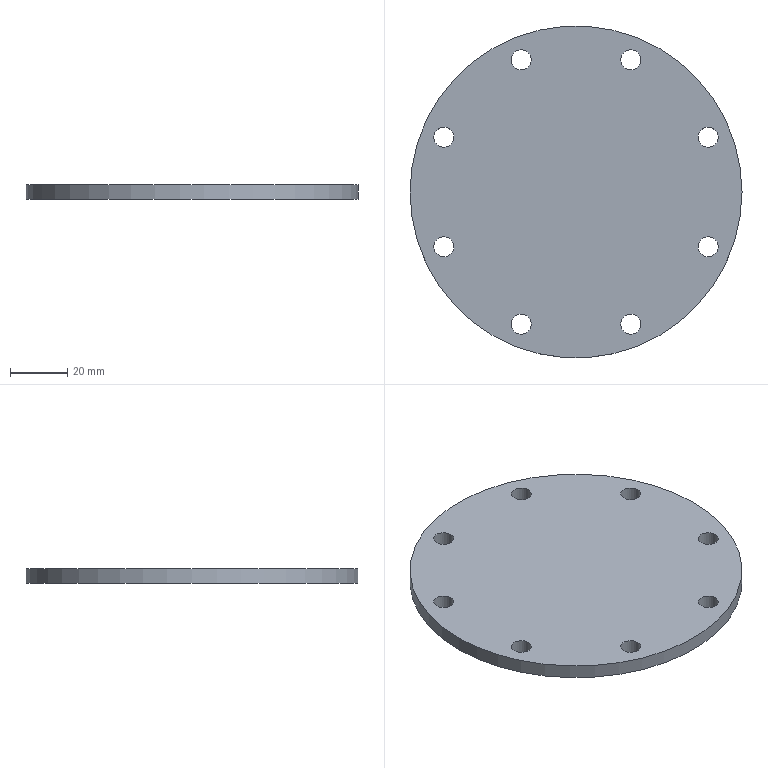Component | NX | CH3404-3 | 1 solid | 11 faces | box 116 x 116 x 5 mm | volume 51302 mm3 | cylinder 9 | plane 2 | commonest cylinder face diameters 7 x8 116 x1
STEP:
#1=CARTESIAN_POINT('',(0.,0.,0.));
#2=DIRECTION('',(0.,0.,1.));
#3=DIRECTION('',(1.,0.,0.));
#4=AXIS2_PLACEMENT_3D('',#1,#2,#3);
#5=CARTESIAN_POINT('',(58.531,0.1057,-1492.003));
#6=VERTEX_POINT('',#5);
#7=CARTESIAN_POINT('',(0.5308,0.1057,-1492.003));
#8=DIRECTION('',(0.,0.,1.));
#9=DIRECTION('',(1.,0.,0.));
#10=AXIS2_PLACEMENT_3D('',#7,#8,#9);
#11=CIRCLE('',#10,58.);
#12=CARTESIAN_POINT('',(0.5308,0.1057,-1492.003));
#13=DIRECTION('',(0.,0.,-1.));
#14=DIRECTION('',(-1.,0.,0.));
#15=AXIS2_PLACEMENT_3D('',#12,#13,#14);
#16=CYLINDRICAL_SURFACE('',#15,58.);
#17=CARTESIAN_POINT('',(9.425,0.));
#18=DIRECTION('',(-1.,0.));
#19=VECTOR('',#18,1.);
#20=LINE('',#17,#19);
#21=(GEOMETRIC_REPRESENTATION_CONTEXT(2)PARAMETRIC_REPRESENTATION_CONTEXT()REPRESENTATION_CONTEXT('',''));
#22=DEFINITIONAL_REPRESENTATION('',(#20),#21);
#23=PCURVE('',#16,#22);
#24=CARTESIAN_POINT('',(0.5308,0.1057,-1492.003));
#25=DIRECTION('',(0.,0.,1.));
#26=DIRECTION('',(1.,0.,0.));
#27=AXIS2_PLACEMENT_3D('',#24,#25,#26);
#28=PLANE('',#27);
#29=CARTESIAN_POINT('',(0.,0.));
#30=DIRECTION('',(1.,0.));
#31=AXIS2_PLACEMENT_2D('',#29,#30);
#32=CIRCLE('',#31,58.);
#33=(GEOMETRIC_REPRESENTATION_CONTEXT(2)PARAMETRIC_REPRESENTATION_CONTEXT()REPRESENTATION_CONTEXT('',''));
#34=DEFINITIONAL_REPRESENTATION('',(#32),#33);
#35=PCURVE('',#28,#34);
#36=SURFACE_CURVE('',#11,(#23,#35),.PCURVE_S1.);
#37=EDGE_CURVE('',#6,#6,#36,.T.);
#38=ORIENTED_EDGE('',*,*,#37,.F.);
#39=CARTESIAN_POINT('',(58.531,0.1057,-1497.003));
#40=VERTEX_POINT('',#39);
#41=CARTESIAN_POINT('',(58.531,0.1057,-1492.003));
#42=CARTESIAN_POINT('',(58.531,0.1057,-1497.003));
#43=B_SPLINE_CURVE_WITH_KNOTS('',1,(#41,#42),.UNSPECIFIED.,.F.,.F.,(2,2),(0.,5.),.PIECEWISE_BEZIER_KNOTS.);
#44=CARTESIAN_POINT('',(9.425,0.));
#45=DIRECTION('',(0.,1.));
#46=VECTOR('',#45,1.);
#47=LINE('',#44,#46);
#48=(GEOMETRIC_REPRESENTATION_CONTEXT(2)PARAMETRIC_REPRESENTATION_CONTEXT()REPRESENTATION_CONTEXT('',''));
#49=DEFINITIONAL_REPRESENTATION('',(#47),#48);
#50=PCURVE('',#16,#49);
#51=CARTESIAN_POINT('',(3.142,0.));
#52=DIRECTION('',(0.,1.));
#53=VECTOR('',#52,1.);
#54=LINE('',#51,#53);
#55=(GEOMETRIC_REPRESENTATION_CONTEXT(2)PARAMETRIC_REPRESENTATION_CONTEXT()REPRESENTATION_CONTEXT('',''));
#56=DEFINITIONAL_REPRESENTATION('',(#54),#55);
#57=PCURVE('',#16,#56);
#58=SEAM_CURVE('',#43,(#50,#57),.PCURVE_S1.);
#59=EDGE_CURVE('',#6,#40,#58,.T.);
#60=ORIENTED_EDGE('',*,*,#59,.T.);
#61=CARTESIAN_POINT('',(0.5308,0.1057,-1497.003));
#62=DIRECTION('',(0.,0.,1.));
#63=DIRECTION('',(1.,0.,0.));
#64=AXIS2_PLACEMENT_3D('',#61,#62,#63);
#65=CIRCLE('',#64,58.);
#66=CARTESIAN_POINT('',(9.425,5.));
#67=DIRECTION('',(-1.,0.));
#68=VECTOR('',#67,1.);
#69=LINE('',#66,#68);
#70=(GEOMETRIC_REPRESENTATION_CONTEXT(2)PARAMETRIC_REPRESENTATION_CONTEXT()REPRESENTATION_CONTEXT('',''));
#71=DEFINITIONAL_REPRESENTATION('',(#69),#70);
#72=PCURVE('',#16,#71);
#73=CARTESIAN_POINT('',(0.5308,0.1057,-1497.003));
#74=DIRECTION('',(0.,0.,1.));
#75=DIRECTION('',(1.,0.,0.));
#76=AXIS2_PLACEMENT_3D('',#73,#74,#75);
#77=PLANE('',#76);
#78=CARTESIAN_POINT('',(0.,0.));
#79=DIRECTION('',(1.,0.));
#80=AXIS2_PLACEMENT_2D('',#78,#79);
#81=CIRCLE('',#80,58.);
#82=(GEOMETRIC_REPRESENTATION_CONTEXT(2)PARAMETRIC_REPRESENTATION_CONTEXT()REPRESENTATION_CONTEXT('',''));
#83=DEFINITIONAL_REPRESENTATION('',(#81),#82);
#84=PCURVE('',#77,#83);
#85=SURFACE_CURVE('',#65,(#72,#84),.PCURVE_S1.);
#86=EDGE_CURVE('',#40,#40,#85,.T.);
#87=ORIENTED_EDGE('',*,*,#86,.T.);
#88=ORIENTED_EDGE('',*,*,#59,.F.);
#89=EDGE_LOOP('',(#38,#60,#87,#88));
#90=FACE_BOUND('',#89,.T.);
#91=ADVANCED_FACE('',(#90),#16,.T.);
#92=CARTESIAN_POINT('',(43.225,-19.028,-1492.003));
#93=VERTEX_POINT('',#92);
#94=CARTESIAN_POINT('',(46.725,-19.028,-1492.003));
#95=DIRECTION('',(0.,0.,-1.));
#96=DIRECTION('',(-1.,0.,0.));
#97=AXIS2_PLACEMENT_3D('',#94,#95,#96);
#98=CIRCLE('',#97,3.5);
#99=CARTESIAN_POINT('',(42.694,-19.134));
#100=CARTESIAN_POINT('',(42.694,-13.072));
#101=CARTESIAN_POINT('',(47.944,-16.103));
#102=CARTESIAN_POINT('',(53.194,-19.134));
#103=CARTESIAN_POINT('',(47.944,-22.165));
#104=CARTESIAN_POINT('',(42.694,-25.196));
#105=CARTESIAN_POINT('',(42.694,-19.134));
#106=(BOUNDED_CURVE()B_SPLINE_CURVE(2,(#99,#100,#101,#102,#103,#104,#105),.UNSPECIFIED.,.T.,.F.)B_SPLINE_CURVE_WITH_KNOTS((1,2,2,2,2,1),(-2.094,0.,2.094,4.189,6.283,8.378),.UNSPECIFIED.)CURVE()GEOMETRIC_REPRESENTATION_ITEM()RATIONAL_B_SPLINE_CURVE((1.,0.5,1.,0.5,1.,0.5,1.))REPRESENTATION_ITEM(''));
#107=(GEOMETRIC_REPRESENTATION_CONTEXT(2)PARAMETRIC_REPRESENTATION_CONTEXT()REPRESENTATION_CONTEXT('',''));
#108=DEFINITIONAL_REPRESENTATION('',(#106),#107);
#109=PCURVE('',#28,#108);
#110=CARTESIAN_POINT('',(46.725,-19.028,-1492.003));
#111=DIRECTION('',(0.,0.,-1.));
#112=DIRECTION('',(-1.,0.,0.));
#113=AXIS2_PLACEMENT_3D('',#110,#111,#112);
#114=CYLINDRICAL_SURFACE('',#113,3.5);
#115=CARTESIAN_POINT('',(0.,0.));
#116=DIRECTION('',(1.,0.));
#117=VECTOR('',#116,1.);
#118=LINE('',#115,#117);
#119=(GEOMETRIC_REPRESENTATION_CONTEXT(2)PARAMETRIC_REPRESENTATION_CONTEXT()REPRESENTATION_CONTEXT('',''));
#120=DEFINITIONAL_REPRESENTATION('',(#118),#119);
#121=PCURVE('',#114,#120);
#122=SURFACE_CURVE('',#98,(#109,#121),.PCURVE_S1.);
#123=EDGE_CURVE('',#93,#93,#122,.T.);
#124=ORIENTED_EDGE('',*,*,#123,.T.);
#125=EDGE_LOOP('',(#124));
#126=FACE_BOUND('',#125,.T.);
#127=CARTESIAN_POINT('',(16.165,-46.088,-1492.003));
#128=VERTEX_POINT('',#127);
#129=CARTESIAN_POINT('',(19.665,-46.088,-1492.003));
#130=DIRECTION('',(0.,0.,-1.));
#131=DIRECTION('',(-1.,0.,0.));
#132=AXIS2_PLACEMENT_3D('',#129,#130,#131);
#133=CIRCLE('',#132,3.5);
#134=CARTESIAN_POINT('',(15.634,-46.194));
#135=CARTESIAN_POINT('',(15.634,-40.132));
#136=CARTESIAN_POINT('',(20.884,-43.163));
#137=CARTESIAN_POINT('',(26.134,-46.194));
#138=CARTESIAN_POINT('',(20.884,-49.225));
#139=CARTESIAN_POINT('',(15.634,-52.256));
#140=CARTESIAN_POINT('',(15.634,-46.194));
#141=(BOUNDED_CURVE()B_SPLINE_CURVE(2,(#134,#135,#136,#137,#138,#139,#140),.UNSPECIFIED.,.T.,.F.)B_SPLINE_CURVE_WITH_KNOTS((1,2,2,2,2,1),(-2.094,0.,2.094,4.189,6.283,8.378),.UNSPECIFIED.)CURVE()GEOMETRIC_REPRESENTATION_ITEM()RATIONAL_B_SPLINE_CURVE((1.,0.5,1.,0.5,1.,0.5,1.))REPRESENTATION_ITEM(''));
#142=(GEOMETRIC_REPRESENTATION_CONTEXT(2)PARAMETRIC_REPRESENTATION_CONTEXT()REPRESENTATION_CONTEXT('',''));
#143=DEFINITIONAL_REPRESENTATION('',(#141),#142);
#144=PCURVE('',#28,#143);
#145=CARTESIAN_POINT('',(19.665,-46.088,-1492.003));
#146=DIRECTION('',(0.,0.,-1.));
#147=DIRECTION('',(-1.,0.,0.));
#148=AXIS2_PLACEMENT_3D('',#145,#146,#147);
#149=CYLINDRICAL_SURFACE('',#148,3.5);
#150=CARTESIAN_POINT('',(0.,0.));
#151=DIRECTION('',(1.,0.));
#152=VECTOR('',#151,1.);
#153=LINE('',#150,#152);
#154=(GEOMETRIC_REPRESENTATION_CONTEXT(2)PARAMETRIC_REPRESENTATION_CONTEXT()REPRESENTATION_CONTEXT('',''));
#155=DEFINITIONAL_REPRESENTATION('',(#153),#154);
#156=PCURVE('',#149,#155);
#157=SURFACE_CURVE('',#133,(#144,#156),.PCURVE_S1.);
#158=EDGE_CURVE('',#128,#128,#157,.T.);
#159=ORIENTED_EDGE('',*,*,#158,.T.);
#160=EDGE_LOOP('',(#159));
#161=FACE_BOUND('',#160,.T.);
#162=CARTESIAN_POINT('',(-22.103,-46.088,-1492.003));
#163=VERTEX_POINT('',#162);
#164=CARTESIAN_POINT('',(-18.603,-46.088,-1492.003));
#165=DIRECTION('',(0.,0.,-1.));
#166=DIRECTION('',(-1.,0.,0.));
#167=AXIS2_PLACEMENT_3D('',#164,#165,#166);
#168=CIRCLE('',#167,3.5);
#169=CARTESIAN_POINT('',(-22.634,-46.194));
#170=CARTESIAN_POINT('',(-22.634,-40.132));
#171=CARTESIAN_POINT('',(-17.384,-43.163));
#172=CARTESIAN_POINT('',(-12.134,-46.194));
#173=CARTESIAN_POINT('',(-17.384,-49.225));
#174=CARTESIAN_POINT('',(-22.634,-52.256));
#175=CARTESIAN_POINT('',(-22.634,-46.194));
#176=(BOUNDED_CURVE()B_SPLINE_CURVE(2,(#169,#170,#171,#172,#173,#174,#175),.UNSPECIFIED.,.T.,.F.)B_SPLINE_CURVE_WITH_KNOTS((1,2,2,2,2,1),(-2.094,0.,2.094,4.189,6.283,8.378),.UNSPECIFIED.)CURVE()GEOMETRIC_REPRESENTATION_ITEM()RATIONAL_B_SPLINE_CURVE((1.,0.5,1.,0.5,1.,0.5,1.))REPRESENTATION_ITEM(''));
#177=(GEOMETRIC_REPRESENTATION_CONTEXT(2)PARAMETRIC_REPRESENTATION_CONTEXT()REPRESENTATION_CONTEXT('',''));
#178=DEFINITIONAL_REPRESENTATION('',(#176),#177);
#179=PCURVE('',#28,#178);
#180=CARTESIAN_POINT('',(-18.603,-46.088,-1492.003));
#181=DIRECTION('',(0.,0.,-1.));
#182=DIRECTION('',(-1.,0.,0.));
#183=AXIS2_PLACEMENT_3D('',#180,#181,#182);
#184=CYLINDRICAL_SURFACE('',#183,3.5);
#185=CARTESIAN_POINT('',(0.,0.));
#186=DIRECTION('',(1.,0.));
#187=VECTOR('',#186,1.);
#188=LINE('',#185,#187);
#189=(GEOMETRIC_REPRESENTATION_CONTEXT(2)PARAMETRIC_REPRESENTATION_CONTEXT()REPRESENTATION_CONTEXT('',''));
#190=DEFINITIONAL_REPRESENTATION('',(#188),#189);
#191=PCURVE('',#184,#190);
#192=SURFACE_CURVE('',#168,(#179,#191),.PCURVE_S1.);
#193=EDGE_CURVE('',#163,#163,#192,.T.);
#194=ORIENTED_EDGE('',*,*,#193,.T.);
#195=EDGE_LOOP('',(#194));
#196=FACE_BOUND('',#195,.T.);
#197=CARTESIAN_POINT('',(-49.163,-19.028,-1492.003));
#198=VERTEX_POINT('',#197);
#199=CARTESIAN_POINT('',(-45.663,-19.028,-1492.003));
#200=DIRECTION('',(0.,0.,-1.));
#201=DIRECTION('',(-1.,0.,0.));
#202=AXIS2_PLACEMENT_3D('',#199,#200,#201);
#203=CIRCLE('',#202,3.5);
#204=CARTESIAN_POINT('',(-49.694,-19.134));
#205=CARTESIAN_POINT('',(-49.694,-13.072));
#206=CARTESIAN_POINT('',(-44.444,-16.103));
#207=CARTESIAN_POINT('',(-39.194,-19.134));
#208=CARTESIAN_POINT('',(-44.444,-22.165));
#209=CARTESIAN_POINT('',(-49.694,-25.196));
#210=CARTESIAN_POINT('',(-49.694,-19.134));
#211=(BOUNDED_CURVE()B_SPLINE_CURVE(2,(#204,#205,#206,#207,#208,#209,#210),.UNSPECIFIED.,.T.,.F.)B_SPLINE_CURVE_WITH_KNOTS((1,2,2,2,2,1),(-2.094,0.,2.094,4.189,6.283,8.378),.UNSPECIFIED.)CURVE()GEOMETRIC_REPRESENTATION_ITEM()RATIONAL_B_SPLINE_CURVE((1.,0.5,1.,0.5,1.,0.5,1.))REPRESENTATION_ITEM(''));
#212=(GEOMETRIC_REPRESENTATION_CONTEXT(2)PARAMETRIC_REPRESENTATION_CONTEXT()REPRESENTATION_CONTEXT('',''));
#213=DEFINITIONAL_REPRESENTATION('',(#211),#212);
#214=PCURVE('',#28,#213);
#215=CARTESIAN_POINT('',(-45.663,-19.028,-1492.003));
#216=DIRECTION('',(0.,0.,-1.));
#217=DIRECTION('',(-1.,0.,0.));
#218=AXIS2_PLACEMENT_3D('',#215,#216,#217);
#219=CYLINDRICAL_SURFACE('',#218,3.5);
#220=CARTESIAN_POINT('',(0.,0.));
#221=DIRECTION('',(1.,0.));
#222=VECTOR('',#221,1.);
#223=LINE('',#220,#222);
#224=(GEOMETRIC_REPRESENTATION_CONTEXT(2)PARAMETRIC_REPRESENTATION_CONTEXT()REPRESENTATION_CONTEXT('',''));
#225=DEFINITIONAL_REPRESENTATION('',(#223),#224);
#226=PCURVE('',#219,#225);
#227=SURFACE_CURVE('',#203,(#214,#226),.PCURVE_S1.);
#228=EDGE_CURVE('',#198,#198,#227,.T.);
#229=ORIENTED_EDGE('',*,*,#228,.T.);
#230=EDGE_LOOP('',(#229));
#231=FACE_BOUND('',#230,.T.);
#232=CARTESIAN_POINT('',(-49.163,19.24,-1492.003));
#233=VERTEX_POINT('',#232);
#234=CARTESIAN_POINT('',(-45.663,19.24,-1492.003));
#235=DIRECTION('',(0.,0.,-1.));
#236=DIRECTION('',(-1.,0.,0.));
#237=AXIS2_PLACEMENT_3D('',#234,#235,#236);
#238=CIRCLE('',#237,3.5);
#239=CARTESIAN_POINT('',(-49.694,19.134));
#240=CARTESIAN_POINT('',(-49.694,25.196));
#241=CARTESIAN_POINT('',(-44.444,22.165));
#242=CARTESIAN_POINT('',(-39.194,19.134));
#243=CARTESIAN_POINT('',(-44.444,16.103));
#244=CARTESIAN_POINT('',(-49.694,13.072));
#245=CARTESIAN_POINT('',(-49.694,19.134));
#246=(BOUNDED_CURVE()B_SPLINE_CURVE(2,(#239,#240,#241,#242,#243,#244,#245),.UNSPECIFIED.,.T.,.F.)B_SPLINE_CURVE_WITH_KNOTS((1,2,2,2,2,1),(-2.094,0.,2.094,4.189,6.283,8.378),.UNSPECIFIED.)CURVE()GEOMETRIC_REPRESENTATION_ITEM()RATIONAL_B_SPLINE_CURVE((1.,0.5,1.,0.5,1.,0.5,1.))REPRESENTATION_ITEM(''));
#247=(GEOMETRIC_REPRESENTATION_CONTEXT(2)PARAMETRIC_REPRESENTATION_CONTEXT()REPRESENTATION_CONTEXT('',''));
#248=DEFINITIONAL_REPRESENTATION('',(#246),#247);
#249=PCURVE('',#28,#248);
#250=CARTESIAN_POINT('',(-45.663,19.24,-1492.003));
#251=DIRECTION('',(0.,0.,-1.));
#252=DIRECTION('',(-1.,0.,0.));
#253=AXIS2_PLACEMENT_3D('',#250,#251,#252);
#254=CYLINDRICAL_SURFACE('',#253,3.5);
#255=CARTESIAN_POINT('',(0.,0.));
#256=DIRECTION('',(1.,0.));
#257=VECTOR('',#256,1.);
#258=LINE('',#255,#257);
#259=(GEOMETRIC_REPRESENTATION_CONTEXT(2)PARAMETRIC_REPRESENTATION_CONTEXT()REPRESENTATION_CONTEXT('',''));
#260=DEFINITIONAL_REPRESENTATION('',(#258),#259);
#261=PCURVE('',#254,#260);
#262=SURFACE_CURVE('',#238,(#249,#261),.PCURVE_S1.);
#263=EDGE_CURVE('',#233,#233,#262,.T.);
#264=ORIENTED_EDGE('',*,*,#263,.T.);
#265=EDGE_LOOP('',(#264));
#266=FACE_BOUND('',#265,.T.);
#267=CARTESIAN_POINT('',(-22.103,46.3,-1492.003));
#268=VERTEX_POINT('',#267);
#269=CARTESIAN_POINT('',(-18.603,46.3,-1492.003));
#270=DIRECTION('',(0.,0.,-1.));
#271=DIRECTION('',(-1.,0.,0.));
#272=AXIS2_PLACEMENT_3D('',#269,#270,#271);
#273=CIRCLE('',#272,3.5);
#274=CARTESIAN_POINT('',(-22.634,46.194));
#275=CARTESIAN_POINT('',(-22.634,52.256));
#276=CARTESIAN_POINT('',(-17.384,49.225));
#277=CARTESIAN_POINT('',(-12.134,46.194));
#278=CARTESIAN_POINT('',(-17.384,43.163));
#279=CARTESIAN_POINT('',(-22.634,40.132));
#280=CARTESIAN_POINT('',(-22.634,46.194));
#281=(BOUNDED_CURVE()B_SPLINE_CURVE(2,(#274,#275,#276,#277,#278,#279,#280),.UNSPECIFIED.,.T.,.F.)B_SPLINE_CURVE_WITH_KNOTS((1,2,2,2,2,1),(-2.094,0.,2.094,4.189,6.283,8.378),.UNSPECIFIED.)CURVE()GEOMETRIC_REPRESENTATION_ITEM()RATIONAL_B_SPLINE_CURVE((1.,0.5,1.,0.5,1.,0.5,1.))REPRESENTATION_ITEM(''));
#282=(GEOMETRIC_REPRESENTATION_CONTEXT(2)PARAMETRIC_REPRESENTATION_CONTEXT()REPRESENTATION_CONTEXT('',''));
#283=DEFINITIONAL_REPRESENTATION('',(#281),#282);
#284=PCURVE('',#28,#283);
#285=CARTESIAN_POINT('',(-18.603,46.3,-1492.003));
#286=DIRECTION('',(0.,0.,-1.));
#287=DIRECTION('',(-1.,0.,0.));
#288=AXIS2_PLACEMENT_3D('',#285,#286,#287);
#289=CYLINDRICAL_SURFACE('',#288,3.5);
#290=CARTESIAN_POINT('',(0.,0.));
#291=DIRECTION('',(1.,0.));
#292=VECTOR('',#291,1.);
#293=LINE('',#290,#292);
#294=(GEOMETRIC_REPRESENTATION_CONTEXT(2)PARAMETRIC_REPRESENTATION_CONTEXT()REPRESENTATION_CONTEXT('',''));
#295=DEFINITIONAL_REPRESENTATION('',(#293),#294);
#296=PCURVE('',#289,#295);
#297=SURFACE_CURVE('',#273,(#284,#296),.PCURVE_S1.);
#298=EDGE_CURVE('',#268,#268,#297,.T.);
#299=ORIENTED_EDGE('',*,*,#298,.T.);
#300=EDGE_LOOP('',(#299));
#301=FACE_BOUND('',#300,.T.);
#302=CARTESIAN_POINT('',(16.165,46.3,-1492.003));
#303=VERTEX_POINT('',#302);
#304=CARTESIAN_POINT('',(19.665,46.3,-1492.003));
#305=DIRECTION('',(0.,0.,-1.));
#306=DIRECTION('',(-1.,0.,0.));
#307=AXIS2_PLACEMENT_3D('',#304,#305,#306);
#308=CIRCLE('',#307,3.5);
#309=CARTESIAN_POINT('',(15.634,46.194));
#310=CARTESIAN_POINT('',(15.634,52.256));
#311=CARTESIAN_POINT('',(20.884,49.225));
#312=CARTESIAN_POINT('',(26.134,46.194));
#313=CARTESIAN_POINT('',(20.884,43.163));
#314=CARTESIAN_POINT('',(15.634,40.132));
#315=CARTESIAN_POINT('',(15.634,46.194));
#316=(BOUNDED_CURVE()B_SPLINE_CURVE(2,(#309,#310,#311,#312,#313,#314,#315),.UNSPECIFIED.,.T.,.F.)B_SPLINE_CURVE_WITH_KNOTS((1,2,2,2,2,1),(-2.094,0.,2.094,4.189,6.283,8.378),.UNSPECIFIED.)CURVE()GEOMETRIC_REPRESENTATION_ITEM()RATIONAL_B_SPLINE_CURVE((1.,0.5,1.,0.5,1.,0.5,1.))REPRESENTATION_ITEM(''));
#317=(GEOMETRIC_REPRESENTATION_CONTEXT(2)PARAMETRIC_REPRESENTATION_CONTEXT()REPRESENTATION_CONTEXT('',''));
#318=DEFINITIONAL_REPRESENTATION('',(#316),#317);
#319=PCURVE('',#28,#318);
#320=CARTESIAN_POINT('',(19.665,46.3,-1492.003));
#321=DIRECTION('',(0.,0.,-1.));
#322=DIRECTION('',(-1.,0.,0.));
#323=AXIS2_PLACEMENT_3D('',#320,#321,#322);
#324=CYLINDRICAL_SURFACE('',#323,3.5);
#325=CARTESIAN_POINT('',(0.,0.));
#326=DIRECTION('',(1.,0.));
#327=VECTOR('',#326,1.);
#328=LINE('',#325,#327);
#329=(GEOMETRIC_REPRESENTATION_CONTEXT(2)PARAMETRIC_REPRESENTATION_CONTEXT()REPRESENTATION_CONTEXT('',''));
#330=DEFINITIONAL_REPRESENTATION('',(#328),#329);
#331=PCURVE('',#324,#330);
#332=SURFACE_CURVE('',#308,(#319,#331),.PCURVE_S1.);
#333=EDGE_CURVE('',#303,#303,#332,.T.);
#334=ORIENTED_EDGE('',*,*,#333,.T.);
#335=EDGE_LOOP('',(#334));
#336=FACE_BOUND('',#335,.T.);
#337=CARTESIAN_POINT('',(43.225,19.24,-1492.003));
#338=VERTEX_POINT('',#337);
#339=CARTESIAN_POINT('',(46.725,19.24,-1492.003));
#340=DIRECTION('',(0.,0.,-1.));
#341=DIRECTION('',(-1.,0.,0.));
#342=AXIS2_PLACEMENT_3D('',#339,#340,#341);
#343=CIRCLE('',#342,3.5);
#344=CARTESIAN_POINT('',(42.694,19.134));
#345=CARTESIAN_POINT('',(42.694,25.196));
#346=CARTESIAN_POINT('',(47.944,22.165));
#347=CARTESIAN_POINT('',(53.194,19.134));
#348=CARTESIAN_POINT('',(47.944,16.103));
#349=CARTESIAN_POINT('',(42.694,13.072));
#350=CARTESIAN_POINT('',(42.694,19.134));
#351=(BOUNDED_CURVE()B_SPLINE_CURVE(2,(#344,#345,#346,#347,#348,#349,#350),.UNSPECIFIED.,.T.,.F.)B_SPLINE_CURVE_WITH_KNOTS((1,2,2,2,2,1),(-2.094,0.,2.094,4.189,6.283,8.378),.UNSPECIFIED.)CURVE()GEOMETRIC_REPRESENTATION_ITEM()RATIONAL_B_SPLINE_CURVE((1.,0.5,1.,0.5,1.,0.5,1.))REPRESENTATION_ITEM(''));
#352=(GEOMETRIC_REPRESENTATION_CONTEXT(2)PARAMETRIC_REPRESENTATION_CONTEXT()REPRESENTATION_CONTEXT('',''));
#353=DEFINITIONAL_REPRESENTATION('',(#351),#352);
#354=PCURVE('',#28,#353);
#355=CARTESIAN_POINT('',(46.725,19.24,-1492.003));
#356=DIRECTION('',(0.,0.,-1.));
#357=DIRECTION('',(-1.,0.,0.));
#358=AXIS2_PLACEMENT_3D('',#355,#356,#357);
#359=CYLINDRICAL_SURFACE('',#358,3.5);
#360=CARTESIAN_POINT('',(0.,0.));
#361=DIRECTION('',(1.,0.));
#362=VECTOR('',#361,1.);
#363=LINE('',#360,#362);
#364=(GEOMETRIC_REPRESENTATION_CONTEXT(2)PARAMETRIC_REPRESENTATION_CONTEXT()REPRESENTATION_CONTEXT('',''));
#365=DEFINITIONAL_REPRESENTATION('',(#363),#364);
#366=PCURVE('',#359,#365);
#367=SURFACE_CURVE('',#343,(#354,#366),.PCURVE_S1.);
#368=EDGE_CURVE('',#338,#338,#367,.T.);
#369=ORIENTED_EDGE('',*,*,#368,.T.);
#370=EDGE_LOOP('',(#369));
#371=FACE_BOUND('',#370,.T.);
#372=ORIENTED_EDGE('',*,*,#37,.T.);
#373=EDGE_LOOP('',(#372));
#374=FACE_BOUND('',#373,.T.);
#375=ADVANCED_FACE('',(#126,#161,#196,#231,#266,#301,#336,#371,#374),#28,.T.);
#376=CARTESIAN_POINT('',(50.225,-19.028,-1497.003));
#377=VERTEX_POINT('',#376);
#378=CARTESIAN_POINT('',(43.225,-19.028,-1497.003));
#379=VERTEX_POINT('',#378);
#380=CARTESIAN_POINT('',(46.725,-19.028,-1497.003));
#381=DIRECTION('',(0.,0.,1.));
#382=DIRECTION('',(1.,0.,0.));
#383=AXIS2_PLACEMENT_3D('',#380,#381,#382);
#384=CIRCLE('',#383,3.5);
#385=CARTESIAN_POINT('',(46.194,-19.134));
#386=DIRECTION('',(1.,0.));
#387=AXIS2_PLACEMENT_2D('',#385,#386);
#388=CIRCLE('',#387,3.5);
#389=(GEOMETRIC_REPRESENTATION_CONTEXT(2)PARAMETRIC_REPRESENTATION_CONTEXT()REPRESENTATION_CONTEXT('',''));
#390=DEFINITIONAL_REPRESENTATION('',(#388),#389);
#391=PCURVE('',#77,#390);
#392=CARTESIAN_POINT('',(3.142,5.));
#393=DIRECTION('',(-1.,0.));
#394=VECTOR('',#393,1.);
#395=LINE('',#392,#394);
#396=(GEOMETRIC_REPRESENTATION_CONTEXT(2)PARAMETRIC_REPRESENTATION_CONTEXT()REPRESENTATION_CONTEXT('',''));
#397=DEFINITIONAL_REPRESENTATION('',(#395),#396);
#398=PCURVE('',#114,#397);
#399=SURFACE_CURVE('',#384,(#391,#398),.PCURVE_S1.);
#400=EDGE_CURVE('',#377,#379,#399,.T.);
#401=ORIENTED_EDGE('',*,*,#400,.T.);
#402=CARTESIAN_POINT('',(46.725,-19.028,-1497.003));
#403=DIRECTION('',(0.,0.,1.));
#404=DIRECTION('',(1.,0.,0.));
#405=AXIS2_PLACEMENT_3D('',#402,#403,#404);
#406=CIRCLE('',#405,3.5);
#407=CARTESIAN_POINT('',(46.194,-19.134));
#408=DIRECTION('',(1.,0.));
#409=AXIS2_PLACEMENT_2D('',#407,#408);
#410=CIRCLE('',#409,3.5);
#411=(GEOMETRIC_REPRESENTATION_CONTEXT(2)PARAMETRIC_REPRESENTATION_CONTEXT()REPRESENTATION_CONTEXT('',''));
#412=DEFINITIONAL_REPRESENTATION('',(#410),#411);
#413=PCURVE('',#77,#412);
#414=CARTESIAN_POINT('',(9.425,5.));
#415=DIRECTION('',(-1.,0.));
#416=VECTOR('',#415,1.);
#417=LINE('',#414,#416);
#418=(GEOMETRIC_REPRESENTATION_CONTEXT(2)PARAMETRIC_REPRESENTATION_CONTEXT()REPRESENTATION_CONTEXT('',''));
#419=DEFINITIONAL_REPRESENTATION('',(#417),#418);
#420=PCURVE('',#114,#419);
#421=SURFACE_CURVE('',#406,(#413,#420),.PCURVE_S1.);
#422=EDGE_CURVE('',#379,#377,#421,.T.);
#423=ORIENTED_EDGE('',*,*,#422,.T.);
#424=EDGE_LOOP('',(#401,#423));
#425=FACE_BOUND('',#424,.T.);
#426=CARTESIAN_POINT('',(23.165,-46.088,-1497.003));
#427=VERTEX_POINT('',#426);
#428=CARTESIAN_POINT('',(16.165,-46.088,-1497.003));
#429=VERTEX_POINT('',#428);
#430=CARTESIAN_POINT('',(19.665,-46.088,-1497.003));
#431=DIRECTION('',(0.,0.,1.));
#432=DIRECTION('',(1.,0.,0.));
#433=AXIS2_PLACEMENT_3D('',#430,#431,#432);
#434=CIRCLE('',#433,3.5);
#435=CARTESIAN_POINT('',(19.134,-46.194));
#436=DIRECTION('',(1.,0.));
#437=AXIS2_PLACEMENT_2D('',#435,#436);
#438=CIRCLE('',#437,3.5);
#439=(GEOMETRIC_REPRESENTATION_CONTEXT(2)PARAMETRIC_REPRESENTATION_CONTEXT()REPRESENTATION_CONTEXT('',''));
#440=DEFINITIONAL_REPRESENTATION('',(#438),#439);
#441=PCURVE('',#77,#440);
#442=CARTESIAN_POINT('',(3.142,5.));
#443=DIRECTION('',(-1.,0.));
#444=VECTOR('',#443,1.);
#445=LINE('',#442,#444);
#446=(GEOMETRIC_REPRESENTATION_CONTEXT(2)PARAMETRIC_REPRESENTATION_CONTEXT()REPRESENTATION_CONTEXT('',''));
#447=DEFINITIONAL_REPRESENTATION('',(#445),#446);
#448=PCURVE('',#149,#447);
#449=SURFACE_CURVE('',#434,(#441,#448),.PCURVE_S1.);
#450=EDGE_CURVE('',#427,#429,#449,.T.);
#451=ORIENTED_EDGE('',*,*,#450,.T.);
#452=CARTESIAN_POINT('',(19.665,-46.088,-1497.003));
#453=DIRECTION('',(0.,0.,1.));
#454=DIRECTION('',(1.,0.,0.));
#455=AXIS2_PLACEMENT_3D('',#452,#453,#454);
#456=CIRCLE('',#455,3.5);
#457=CARTESIAN_POINT('',(19.134,-46.194));
#458=DIRECTION('',(1.,0.));
#459=AXIS2_PLACEMENT_2D('',#457,#458);
#460=CIRCLE('',#459,3.5);
#461=(GEOMETRIC_REPRESENTATION_CONTEXT(2)PARAMETRIC_REPRESENTATION_CONTEXT()REPRESENTATION_CONTEXT('',''));
#462=DEFINITIONAL_REPRESENTATION('',(#460),#461);
#463=PCURVE('',#77,#462);
#464=CARTESIAN_POINT('',(9.425,5.));
#465=DIRECTION('',(-1.,0.));
#466=VECTOR('',#465,1.);
#467=LINE('',#464,#466);
#468=(GEOMETRIC_REPRESENTATION_CONTEXT(2)PARAMETRIC_REPRESENTATION_CONTEXT()REPRESENTATION_CONTEXT('',''));
#469=DEFINITIONAL_REPRESENTATION('',(#467),#468);
#470=PCURVE('',#149,#469);
#471=SURFACE_CURVE('',#456,(#463,#470),.PCURVE_S1.);
#472=EDGE_CURVE('',#429,#427,#471,.T.);
#473=ORIENTED_EDGE('',*,*,#472,.T.);
#474=EDGE_LOOP('',(#451,#473));
#475=FACE_BOUND('',#474,.T.);
#476=CARTESIAN_POINT('',(-15.103,-46.088,-1497.003));
#477=VERTEX_POINT('',#476);
#478=CARTESIAN_POINT('',(-22.103,-46.088,-1497.003));
#479=VERTEX_POINT('',#478);
#480=CARTESIAN_POINT('',(-18.603,-46.088,-1497.003));
#481=DIRECTION('',(0.,0.,1.));
#482=DIRECTION('',(1.,0.,0.));
#483=AXIS2_PLACEMENT_3D('',#480,#481,#482);
#484=CIRCLE('',#483,3.5);
#485=CARTESIAN_POINT('',(-19.134,-46.194));
#486=DIRECTION('',(1.,0.));
#487=AXIS2_PLACEMENT_2D('',#485,#486);
#488=CIRCLE('',#487,3.5);
#489=(GEOMETRIC_REPRESENTATION_CONTEXT(2)PARAMETRIC_REPRESENTATION_CONTEXT()REPRESENTATION_CONTEXT('',''));
#490=DEFINITIONAL_REPRESENTATION('',(#488),#489);
#491=PCURVE('',#77,#490);
#492=CARTESIAN_POINT('',(3.142,5.));
#493=DIRECTION('',(-1.,0.));
#494=VECTOR('',#493,1.);
#495=LINE('',#492,#494);
#496=(GEOMETRIC_REPRESENTATION_CONTEXT(2)PARAMETRIC_REPRESENTATION_CONTEXT()REPRESENTATION_CONTEXT('',''));
#497=DEFINITIONAL_REPRESENTATION('',(#495),#496);
#498=PCURVE('',#184,#497);
#499=SURFACE_CURVE('',#484,(#491,#498),.PCURVE_S1.);
#500=EDGE_CURVE('',#477,#479,#499,.T.);
#501=ORIENTED_EDGE('',*,*,#500,.T.);
#502=CARTESIAN_POINT('',(-18.603,-46.088,-1497.003));
#503=DIRECTION('',(0.,0.,1.));
#504=DIRECTION('',(1.,0.,0.));
#505=AXIS2_PLACEMENT_3D('',#502,#503,#504);
#506=CIRCLE('',#505,3.5);
#507=CARTESIAN_POINT('',(-19.134,-46.194));
#508=DIRECTION('',(1.,0.));
#509=AXIS2_PLACEMENT_2D('',#507,#508);
#510=CIRCLE('',#509,3.5);
#511=(GEOMETRIC_REPRESENTATION_CONTEXT(2)PARAMETRIC_REPRESENTATION_CONTEXT()REPRESENTATION_CONTEXT('',''));
#512=DEFINITIONAL_REPRESENTATION('',(#510),#511);
#513=PCURVE('',#77,#512);
#514=CARTESIAN_POINT('',(9.425,5.));
#515=DIRECTION('',(-1.,0.));
#516=VECTOR('',#515,1.);
#517=LINE('',#514,#516);
#518=(GEOMETRIC_REPRESENTATION_CONTEXT(2)PARAMETRIC_REPRESENTATION_CONTEXT()REPRESENTATION_CONTEXT('',''));
#519=DEFINITIONAL_REPRESENTATION('',(#517),#518);
#520=PCURVE('',#184,#519);
#521=SURFACE_CURVE('',#506,(#513,#520),.PCURVE_S1.);
#522=EDGE_CURVE('',#479,#477,#521,.T.);
#523=ORIENTED_EDGE('',*,*,#522,.T.);
#524=EDGE_LOOP('',(#501,#523));
#525=FACE_BOUND('',#524,.T.);
#526=CARTESIAN_POINT('',(-42.163,-19.028,-1497.003));
#527=VERTEX_POINT('',#526);
#528=CARTESIAN_POINT('',(-49.163,-19.028,-1497.003));
#529=VERTEX_POINT('',#528);
#530=CARTESIAN_POINT('',(-45.663,-19.028,-1497.003));
#531=DIRECTION('',(0.,0.,1.));
#532=DIRECTION('',(1.,0.,0.));
#533=AXIS2_PLACEMENT_3D('',#530,#531,#532);
#534=CIRCLE('',#533,3.5);
#535=CARTESIAN_POINT('',(-46.194,-19.134));
#536=DIRECTION('',(1.,0.));
#537=AXIS2_PLACEMENT_2D('',#535,#536);
#538=CIRCLE('',#537,3.5);
#539=(GEOMETRIC_REPRESENTATION_CONTEXT(2)PARAMETRIC_REPRESENTATION_CONTEXT()REPRESENTATION_CONTEXT('',''));
#540=DEFINITIONAL_REPRESENTATION('',(#538),#539);
#541=PCURVE('',#77,#540);
#542=CARTESIAN_POINT('',(3.142,5.));
#543=DIRECTION('',(-1.,0.));
#544=VECTOR('',#543,1.);
#545=LINE('',#542,#544);
#546=(GEOMETRIC_REPRESENTATION_CONTEXT(2)PARAMETRIC_REPRESENTATION_CONTEXT()REPRESENTATION_CONTEXT('',''));
#547=DEFINITIONAL_REPRESENTATION('',(#545),#546);
#548=PCURVE('',#219,#547);
#549=SURFACE_CURVE('',#534,(#541,#548),.PCURVE_S1.);
#550=EDGE_CURVE('',#527,#529,#549,.T.);
#551=ORIENTED_EDGE('',*,*,#550,.T.);
#552=CARTESIAN_POINT('',(-45.663,-19.028,-1497.003));
#553=DIRECTION('',(0.,0.,1.));
#554=DIRECTION('',(1.,0.,0.));
#555=AXIS2_PLACEMENT_3D('',#552,#553,#554);
#556=CIRCLE('',#555,3.5);
#557=CARTESIAN_POINT('',(-46.194,-19.134));
#558=DIRECTION('',(1.,0.));
#559=AXIS2_PLACEMENT_2D('',#557,#558);
#560=CIRCLE('',#559,3.5);
#561=(GEOMETRIC_REPRESENTATION_CONTEXT(2)PARAMETRIC_REPRESENTATION_CONTEXT()REPRESENTATION_CONTEXT('',''));
#562=DEFINITIONAL_REPRESENTATION('',(#560),#561);
#563=PCURVE('',#77,#562);
#564=CARTESIAN_POINT('',(9.425,5.));
#565=DIRECTION('',(-1.,0.));
#566=VECTOR('',#565,1.);
#567=LINE('',#564,#566);
#568=(GEOMETRIC_REPRESENTATION_CONTEXT(2)PARAMETRIC_REPRESENTATION_CONTEXT()REPRESENTATION_CONTEXT('',''));
#569=DEFINITIONAL_REPRESENTATION('',(#567),#568);
#570=PCURVE('',#219,#569);
#571=SURFACE_CURVE('',#556,(#563,#570),.PCURVE_S1.);
#572=EDGE_CURVE('',#529,#527,#571,.T.);
#573=ORIENTED_EDGE('',*,*,#572,.T.);
#574=EDGE_LOOP('',(#551,#573));
#575=FACE_BOUND('',#574,.T.);
#576=CARTESIAN_POINT('',(-42.163,19.24,-1497.003));
#577=VERTEX_POINT('',#576);
#578=CARTESIAN_POINT('',(-49.163,19.24,-1497.003));
#579=VERTEX_POINT('',#578);
#580=CARTESIAN_POINT('',(-45.663,19.24,-1497.003));
#581=DIRECTION('',(0.,0.,1.));
#582=DIRECTION('',(1.,0.,0.));
#583=AXIS2_PLACEMENT_3D('',#580,#581,#582);
#584=CIRCLE('',#583,3.5);
#585=CARTESIAN_POINT('',(-46.194,19.134));
#586=DIRECTION('',(1.,0.));
#587=AXIS2_PLACEMENT_2D('',#585,#586);
#588=CIRCLE('',#587,3.5);
#589=(GEOMETRIC_REPRESENTATION_CONTEXT(2)PARAMETRIC_REPRESENTATION_CONTEXT()REPRESENTATION_CONTEXT('',''));
#590=DEFINITIONAL_REPRESENTATION('',(#588),#589);
#591=PCURVE('',#77,#590);
#592=CARTESIAN_POINT('',(3.142,5.));
#593=DIRECTION('',(-1.,0.));
#594=VECTOR('',#593,1.);
#595=LINE('',#592,#594);
#596=(GEOMETRIC_REPRESENTATION_CONTEXT(2)PARAMETRIC_REPRESENTATION_CONTEXT()REPRESENTATION_CONTEXT('',''));
#597=DEFINITIONAL_REPRESENTATION('',(#595),#596);
#598=PCURVE('',#254,#597);
#599=SURFACE_CURVE('',#584,(#591,#598),.PCURVE_S1.);
#600=EDGE_CURVE('',#577,#579,#599,.T.);
#601=ORIENTED_EDGE('',*,*,#600,.T.);
#602=CARTESIAN_POINT('',(-45.663,19.24,-1497.003));
#603=DIRECTION('',(0.,0.,1.));
#604=DIRECTION('',(1.,0.,0.));
#605=AXIS2_PLACEMENT_3D('',#602,#603,#604);
#606=CIRCLE('',#605,3.5);
#607=CARTESIAN_POINT('',(-46.194,19.134));
#608=DIRECTION('',(1.,0.));
#609=AXIS2_PLACEMENT_2D('',#607,#608);
#610=CIRCLE('',#609,3.5);
#611=(GEOMETRIC_REPRESENTATION_CONTEXT(2)PARAMETRIC_REPRESENTATION_CONTEXT()REPRESENTATION_CONTEXT('',''));
#612=DEFINITIONAL_REPRESENTATION('',(#610),#611);
#613=PCURVE('',#77,#612);
#614=CARTESIAN_POINT('',(9.425,5.));
#615=DIRECTION('',(-1.,0.));
#616=VECTOR('',#615,1.);
#617=LINE('',#614,#616);
#618=(GEOMETRIC_REPRESENTATION_CONTEXT(2)PARAMETRIC_REPRESENTATION_CONTEXT()REPRESENTATION_CONTEXT('',''));
#619=DEFINITIONAL_REPRESENTATION('',(#617),#618);
#620=PCURVE('',#254,#619);
#621=SURFACE_CURVE('',#606,(#613,#620),.PCURVE_S1.);
#622=EDGE_CURVE('',#579,#577,#621,.T.);
#623=ORIENTED_EDGE('',*,*,#622,.T.);
#624=EDGE_LOOP('',(#601,#623));
#625=FACE_BOUND('',#624,.T.);
#626=CARTESIAN_POINT('',(-15.103,46.3,-1497.003));
#627=VERTEX_POINT('',#626);
#628=CARTESIAN_POINT('',(-22.103,46.3,-1497.003));
#629=VERTEX_POINT('',#628);
#630=CARTESIAN_POINT('',(-18.603,46.3,-1497.003));
#631=DIRECTION('',(0.,0.,1.));
#632=DIRECTION('',(1.,0.,0.));
#633=AXIS2_PLACEMENT_3D('',#630,#631,#632);
#634=CIRCLE('',#633,3.5);
#635=CARTESIAN_POINT('',(-19.134,46.194));
#636=DIRECTION('',(1.,0.));
#637=AXIS2_PLACEMENT_2D('',#635,#636);
#638=CIRCLE('',#637,3.5);
#639=(GEOMETRIC_REPRESENTATION_CONTEXT(2)PARAMETRIC_REPRESENTATION_CONTEXT()REPRESENTATION_CONTEXT('',''));
#640=DEFINITIONAL_REPRESENTATION('',(#638),#639);
#641=PCURVE('',#77,#640);
#642=CARTESIAN_POINT('',(3.142,5.));
#643=DIRECTION('',(-1.,0.));
#644=VECTOR('',#643,1.);
#645=LINE('',#642,#644);
#646=(GEOMETRIC_REPRESENTATION_CONTEXT(2)PARAMETRIC_REPRESENTATION_CONTEXT()REPRESENTATION_CONTEXT('',''));
#647=DEFINITIONAL_REPRESENTATION('',(#645),#646);
#648=PCURVE('',#289,#647);
#649=SURFACE_CURVE('',#634,(#641,#648),.PCURVE_S1.);
#650=EDGE_CURVE('',#627,#629,#649,.T.);
#651=ORIENTED_EDGE('',*,*,#650,.T.);
#652=CARTESIAN_POINT('',(-18.603,46.3,-1497.003));
#653=DIRECTION('',(0.,0.,1.));
#654=DIRECTION('',(1.,0.,0.));
#655=AXIS2_PLACEMENT_3D('',#652,#653,#654);
#656=CIRCLE('',#655,3.5);
#657=CARTESIAN_POINT('',(-19.134,46.194));
#658=DIRECTION('',(1.,0.));
#659=AXIS2_PLACEMENT_2D('',#657,#658);
#660=CIRCLE('',#659,3.5);
#661=(GEOMETRIC_REPRESENTATION_CONTEXT(2)PARAMETRIC_REPRESENTATION_CONTEXT()REPRESENTATION_CONTEXT('',''));
#662=DEFINITIONAL_REPRESENTATION('',(#660),#661);
#663=PCURVE('',#77,#662);
#664=CARTESIAN_POINT('',(9.425,5.));
#665=DIRECTION('',(-1.,0.));
#666=VECTOR('',#665,1.);
#667=LINE('',#664,#666);
#668=(GEOMETRIC_REPRESENTATION_CONTEXT(2)PARAMETRIC_REPRESENTATION_CONTEXT()REPRESENTATION_CONTEXT('',''));
#669=DEFINITIONAL_REPRESENTATION('',(#667),#668);
#670=PCURVE('',#289,#669);
#671=SURFACE_CURVE('',#656,(#663,#670),.PCURVE_S1.);
#672=EDGE_CURVE('',#629,#627,#671,.T.);
#673=ORIENTED_EDGE('',*,*,#672,.T.);
#674=EDGE_LOOP('',(#651,#673));
#675=FACE_BOUND('',#674,.T.);
#676=CARTESIAN_POINT('',(23.165,46.3,-1497.003));
#677=VERTEX_POINT('',#676);
#678=CARTESIAN_POINT('',(16.165,46.3,-1497.003));
#679=VERTEX_POINT('',#678);
#680=CARTESIAN_POINT('',(19.665,46.3,-1497.003));
#681=DIRECTION('',(0.,0.,1.));
#682=DIRECTION('',(1.,0.,0.));
#683=AXIS2_PLACEMENT_3D('',#680,#681,#682);
#684=CIRCLE('',#683,3.5);
#685=CARTESIAN_POINT('',(19.134,46.194));
#686=DIRECTION('',(1.,0.));
#687=AXIS2_PLACEMENT_2D('',#685,#686);
#688=CIRCLE('',#687,3.5);
#689=(GEOMETRIC_REPRESENTATION_CONTEXT(2)PARAMETRIC_REPRESENTATION_CONTEXT()REPRESENTATION_CONTEXT('',''));
#690=DEFINITIONAL_REPRESENTATION('',(#688),#689);
#691=PCURVE('',#77,#690);
#692=CARTESIAN_POINT('',(3.142,5.));
#693=DIRECTION('',(-1.,0.));
#694=VECTOR('',#693,1.);
#695=LINE('',#692,#694);
#696=(GEOMETRIC_REPRESENTATION_CONTEXT(2)PARAMETRIC_REPRESENTATION_CONTEXT()REPRESENTATION_CONTEXT('',''));
#697=DEFINITIONAL_REPRESENTATION('',(#695),#696);
#698=PCURVE('',#324,#697);
#699=SURFACE_CURVE('',#684,(#691,#698),.PCURVE_S1.);
#700=EDGE_CURVE('',#677,#679,#699,.T.);
#701=ORIENTED_EDGE('',*,*,#700,.T.);
#702=CARTESIAN_POINT('',(19.665,46.3,-1497.003));
#703=DIRECTION('',(0.,0.,1.));
#704=DIRECTION('',(1.,0.,0.));
#705=AXIS2_PLACEMENT_3D('',#702,#703,#704);
#706=CIRCLE('',#705,3.5);
#707=CARTESIAN_POINT('',(19.134,46.194));
#708=DIRECTION('',(1.,0.));
#709=AXIS2_PLACEMENT_2D('',#707,#708);
#710=CIRCLE('',#709,3.5);
#711=(GEOMETRIC_REPRESENTATION_CONTEXT(2)PARAMETRIC_REPRESENTATION_CONTEXT()REPRESENTATION_CONTEXT('',''));
#712=DEFINITIONAL_REPRESENTATION('',(#710),#711);
#713=PCURVE('',#77,#712);
#714=CARTESIAN_POINT('',(9.425,5.));
#715=DIRECTION('',(-1.,0.));
#716=VECTOR('',#715,1.);
#717=LINE('',#714,#716);
#718=(GEOMETRIC_REPRESENTATION_CONTEXT(2)PARAMETRIC_REPRESENTATION_CONTEXT()REPRESENTATION_CONTEXT('',''));
#719=DEFINITIONAL_REPRESENTATION('',(#717),#718);
#720=PCURVE('',#324,#719);
#721=SURFACE_CURVE('',#706,(#713,#720),.PCURVE_S1.);
#722=EDGE_CURVE('',#679,#677,#721,.T.);
#723=ORIENTED_EDGE('',*,*,#722,.T.);
#724=EDGE_LOOP('',(#701,#723));
#725=FACE_BOUND('',#724,.T.);
#726=CARTESIAN_POINT('',(50.225,19.24,-1497.003));
#727=VERTEX_POINT('',#726);
#728=CARTESIAN_POINT('',(43.225,19.24,-1497.003));
#729=VERTEX_POINT('',#728);
#730=CARTESIAN_POINT('',(46.725,19.24,-1497.003));
#731=DIRECTION('',(0.,0.,1.));
#732=DIRECTION('',(1.,0.,0.));
#733=AXIS2_PLACEMENT_3D('',#730,#731,#732);
#734=CIRCLE('',#733,3.5);
#735=CARTESIAN_POINT('',(46.194,19.134));
#736=DIRECTION('',(1.,0.));
#737=AXIS2_PLACEMENT_2D('',#735,#736);
#738=CIRCLE('',#737,3.5);
#739=(GEOMETRIC_REPRESENTATION_CONTEXT(2)PARAMETRIC_REPRESENTATION_CONTEXT()REPRESENTATION_CONTEXT('',''));
#740=DEFINITIONAL_REPRESENTATION('',(#738),#739);
#741=PCURVE('',#77,#740);
#742=CARTESIAN_POINT('',(3.142,5.));
#743=DIRECTION('',(-1.,0.));
#744=VECTOR('',#743,1.);
#745=LINE('',#742,#744);
#746=(GEOMETRIC_REPRESENTATION_CONTEXT(2)PARAMETRIC_REPRESENTATION_CONTEXT()REPRESENTATION_CONTEXT('',''));
#747=DEFINITIONAL_REPRESENTATION('',(#745),#746);
#748=PCURVE('',#359,#747);
#749=SURFACE_CURVE('',#734,(#741,#748),.PCURVE_S1.);
#750=EDGE_CURVE('',#727,#729,#749,.T.);
#751=ORIENTED_EDGE('',*,*,#750,.T.);
#752=CARTESIAN_POINT('',(46.725,19.24,-1497.003));
#753=DIRECTION('',(0.,0.,1.));
#754=DIRECTION('',(1.,0.,0.));
#755=AXIS2_PLACEMENT_3D('',#752,#753,#754);
#756=CIRCLE('',#755,3.5);
#757=CARTESIAN_POINT('',(46.194,19.134));
#758=DIRECTION('',(1.,0.));
#759=AXIS2_PLACEMENT_2D('',#757,#758);
#760=CIRCLE('',#759,3.5);
#761=(GEOMETRIC_REPRESENTATION_CONTEXT(2)PARAMETRIC_REPRESENTATION_CONTEXT()REPRESENTATION_CONTEXT('',''));
#762=DEFINITIONAL_REPRESENTATION('',(#760),#761);
#763=PCURVE('',#77,#762);
#764=CARTESIAN_POINT('',(9.425,5.));
#765=DIRECTION('',(-1.,0.));
#766=VECTOR('',#765,1.);
#767=LINE('',#764,#766);
#768=(GEOMETRIC_REPRESENTATION_CONTEXT(2)PARAMETRIC_REPRESENTATION_CONTEXT()REPRESENTATION_CONTEXT('',''));
#769=DEFINITIONAL_REPRESENTATION('',(#767),#768);
#770=PCURVE('',#359,#769);
#771=SURFACE_CURVE('',#756,(#763,#770),.PCURVE_S1.);
#772=EDGE_CURVE('',#729,#727,#771,.T.);
#773=ORIENTED_EDGE('',*,*,#772,.T.);
#774=EDGE_LOOP('',(#751,#773));
#775=FACE_BOUND('',#774,.T.);
#776=ORIENTED_EDGE('',*,*,#86,.F.);
#777=EDGE_LOOP('',(#776));
#778=FACE_BOUND('',#777,.T.);
#779=ADVANCED_FACE('',(#425,#475,#525,#575,#625,#675,#725,#775,#778),#77,.F.);
#780=ORIENTED_EDGE('',*,*,#368,.T.);
#781=CARTESIAN_POINT('',(43.225,19.24,-1492.003));
#782=CARTESIAN_POINT('',(43.225,19.24,-1497.003));
#783=B_SPLINE_CURVE_WITH_KNOTS('',1,(#781,#782),.UNSPECIFIED.,.F.,.F.,(2,2),(0.,5.),.PIECEWISE_BEZIER_KNOTS.);
#784=CARTESIAN_POINT('',(6.283,0.));
#785=DIRECTION('',(0.,1.));
#786=VECTOR('',#785,1.);
#787=LINE('',#784,#786);
#788=(GEOMETRIC_REPRESENTATION_CONTEXT(2)PARAMETRIC_REPRESENTATION_CONTEXT()REPRESENTATION_CONTEXT('',''));
#789=DEFINITIONAL_REPRESENTATION('',(#787),#788);
#790=PCURVE('',#359,#789);
#791=CARTESIAN_POINT('',(0.,0.));
#792=DIRECTION('',(0.,1.));
#793=VECTOR('',#792,1.);
#794=LINE('',#791,#793);
#795=(GEOMETRIC_REPRESENTATION_CONTEXT(2)PARAMETRIC_REPRESENTATION_CONTEXT()REPRESENTATION_CONTEXT('',''));
#796=DEFINITIONAL_REPRESENTATION('',(#794),#795);
#797=PCURVE('',#359,#796);
#798=SEAM_CURVE('',#783,(#790,#797),.PCURVE_S1.);
#799=EDGE_CURVE('',#338,#729,#798,.T.);
#800=ORIENTED_EDGE('',*,*,#799,.T.);
#801=ORIENTED_EDGE('',*,*,#772,.T.);
#802=ORIENTED_EDGE('',*,*,#750,.T.);
#803=ORIENTED_EDGE('',*,*,#799,.F.);
#804=EDGE_LOOP('',(#780,#800,#801,#802,#803));
#805=FACE_BOUND('',#804,.F.);
#806=ADVANCED_FACE('',(#805),#359,.F.);
#807=ORIENTED_EDGE('',*,*,#333,.T.);
#808=CARTESIAN_POINT('',(16.165,46.3,-1492.003));
#809=CARTESIAN_POINT('',(16.165,46.3,-1497.003));
#810=B_SPLINE_CURVE_WITH_KNOTS('',1,(#808,#809),.UNSPECIFIED.,.F.,.F.,(2,2),(0.,5.),.PIECEWISE_BEZIER_KNOTS.);
#811=CARTESIAN_POINT('',(6.283,0.));
#812=DIRECTION('',(0.,1.));
#813=VECTOR('',#812,1.);
#814=LINE('',#811,#813);
#815=(GEOMETRIC_REPRESENTATION_CONTEXT(2)PARAMETRIC_REPRESENTATION_CONTEXT()REPRESENTATION_CONTEXT('',''));
#816=DEFINITIONAL_REPRESENTATION('',(#814),#815);
#817=PCURVE('',#324,#816);
#818=CARTESIAN_POINT('',(0.,0.));
#819=DIRECTION('',(0.,1.));
#820=VECTOR('',#819,1.);
#821=LINE('',#818,#820);
#822=(GEOMETRIC_REPRESENTATION_CONTEXT(2)PARAMETRIC_REPRESENTATION_CONTEXT()REPRESENTATION_CONTEXT('',''));
#823=DEFINITIONAL_REPRESENTATION('',(#821),#822);
#824=PCURVE('',#324,#823);
#825=SEAM_CURVE('',#810,(#817,#824),.PCURVE_S1.);
#826=EDGE_CURVE('',#303,#679,#825,.T.);
#827=ORIENTED_EDGE('',*,*,#826,.T.);
#828=ORIENTED_EDGE('',*,*,#722,.T.);
#829=ORIENTED_EDGE('',*,*,#700,.T.);
#830=ORIENTED_EDGE('',*,*,#826,.F.);
#831=EDGE_LOOP('',(#807,#827,#828,#829,#830));
#832=FACE_BOUND('',#831,.F.);
#833=ADVANCED_FACE('',(#832),#324,.F.);
#834=ORIENTED_EDGE('',*,*,#298,.T.);
#835=CARTESIAN_POINT('',(-22.103,46.3,-1492.003));
#836=CARTESIAN_POINT('',(-22.103,46.3,-1497.003));
#837=B_SPLINE_CURVE_WITH_KNOTS('',1,(#835,#836),.UNSPECIFIED.,.F.,.F.,(2,2),(0.,5.),.PIECEWISE_BEZIER_KNOTS.);
#838=CARTESIAN_POINT('',(6.283,0.));
#839=DIRECTION('',(0.,1.));
#840=VECTOR('',#839,1.);
#841=LINE('',#838,#840);
#842=(GEOMETRIC_REPRESENTATION_CONTEXT(2)PARAMETRIC_REPRESENTATION_CONTEXT()REPRESENTATION_CONTEXT('',''));
#843=DEFINITIONAL_REPRESENTATION('',(#841),#842);
#844=PCURVE('',#289,#843);
#845=CARTESIAN_POINT('',(0.,0.));
#846=DIRECTION('',(0.,1.));
#847=VECTOR('',#846,1.);
#848=LINE('',#845,#847);
#849=(GEOMETRIC_REPRESENTATION_CONTEXT(2)PARAMETRIC_REPRESENTATION_CONTEXT()REPRESENTATION_CONTEXT('',''));
#850=DEFINITIONAL_REPRESENTATION('',(#848),#849);
#851=PCURVE('',#289,#850);
#852=SEAM_CURVE('',#837,(#844,#851),.PCURVE_S1.);
#853=EDGE_CURVE('',#268,#629,#852,.T.);
#854=ORIENTED_EDGE('',*,*,#853,.T.);
#855=ORIENTED_EDGE('',*,*,#672,.T.);
#856=ORIENTED_EDGE('',*,*,#650,.T.);
#857=ORIENTED_EDGE('',*,*,#853,.F.);
#858=EDGE_LOOP('',(#834,#854,#855,#856,#857));
#859=FACE_BOUND('',#858,.F.);
#860=ADVANCED_FACE('',(#859),#289,.F.);
#861=ORIENTED_EDGE('',*,*,#263,.T.);
#862=CARTESIAN_POINT('',(-49.163,19.24,-1492.003));
#863=CARTESIAN_POINT('',(-49.163,19.24,-1497.003));
#864=B_SPLINE_CURVE_WITH_KNOTS('',1,(#862,#863),.UNSPECIFIED.,.F.,.F.,(2,2),(0.,5.),.PIECEWISE_BEZIER_KNOTS.);
#865=CARTESIAN_POINT('',(6.283,0.));
#866=DIRECTION('',(0.,1.));
#867=VECTOR('',#866,1.);
#868=LINE('',#865,#867);
#869=(GEOMETRIC_REPRESENTATION_CONTEXT(2)PARAMETRIC_REPRESENTATION_CONTEXT()REPRESENTATION_CONTEXT('',''));
#870=DEFINITIONAL_REPRESENTATION('',(#868),#869);
#871=PCURVE('',#254,#870);
#872=CARTESIAN_POINT('',(0.,0.));
#873=DIRECTION('',(0.,1.));
#874=VECTOR('',#873,1.);
#875=LINE('',#872,#874);
#876=(GEOMETRIC_REPRESENTATION_CONTEXT(2)PARAMETRIC_REPRESENTATION_CONTEXT()REPRESENTATION_CONTEXT('',''));
#877=DEFINITIONAL_REPRESENTATION('',(#875),#876);
#878=PCURVE('',#254,#877);
#879=SEAM_CURVE('',#864,(#871,#878),.PCURVE_S1.);
#880=EDGE_CURVE('',#233,#579,#879,.T.);
#881=ORIENTED_EDGE('',*,*,#880,.T.);
#882=ORIENTED_EDGE('',*,*,#622,.T.);
#883=ORIENTED_EDGE('',*,*,#600,.T.);
#884=ORIENTED_EDGE('',*,*,#880,.F.);
#885=EDGE_LOOP('',(#861,#881,#882,#883,#884));
#886=FACE_BOUND('',#885,.F.);
#887=ADVANCED_FACE('',(#886),#254,.F.);
#888=ORIENTED_EDGE('',*,*,#228,.T.);
#889=CARTESIAN_POINT('',(-49.163,-19.028,-1492.003));
#890=CARTESIAN_POINT('',(-49.163,-19.028,-1497.003));
#891=B_SPLINE_CURVE_WITH_KNOTS('',1,(#889,#890),.UNSPECIFIED.,.F.,.F.,(2,2),(0.,5.),.PIECEWISE_BEZIER_KNOTS.);
#892=CARTESIAN_POINT('',(6.283,0.));
#893=DIRECTION('',(0.,1.));
#894=VECTOR('',#893,1.);
#895=LINE('',#892,#894);
#896=(GEOMETRIC_REPRESENTATION_CONTEXT(2)PARAMETRIC_REPRESENTATION_CONTEXT()REPRESENTATION_CONTEXT('',''));
#897=DEFINITIONAL_REPRESENTATION('',(#895),#896);
#898=PCURVE('',#219,#897);
#899=CARTESIAN_POINT('',(0.,0.));
#900=DIRECTION('',(0.,1.));
#901=VECTOR('',#900,1.);
#902=LINE('',#899,#901);
#903=(GEOMETRIC_REPRESENTATION_CONTEXT(2)PARAMETRIC_REPRESENTATION_CONTEXT()REPRESENTATION_CONTEXT('',''));
#904=DEFINITIONAL_REPRESENTATION('',(#902),#903);
#905=PCURVE('',#219,#904);
#906=SEAM_CURVE('',#891,(#898,#905),.PCURVE_S1.);
#907=EDGE_CURVE('',#198,#529,#906,.T.);
#908=ORIENTED_EDGE('',*,*,#907,.T.);
#909=ORIENTED_EDGE('',*,*,#572,.T.);
#910=ORIENTED_EDGE('',*,*,#550,.T.);
#911=ORIENTED_EDGE('',*,*,#907,.F.);
#912=EDGE_LOOP('',(#888,#908,#909,#910,#911));
#913=FACE_BOUND('',#912,.F.);
#914=ADVANCED_FACE('',(#913),#219,.F.);
#915=ORIENTED_EDGE('',*,*,#193,.T.);
#916=CARTESIAN_POINT('',(-22.103,-46.088,-1492.003));
#917=CARTESIAN_POINT('',(-22.103,-46.088,-1497.003));
#918=B_SPLINE_CURVE_WITH_KNOTS('',1,(#916,#917),.UNSPECIFIED.,.F.,.F.,(2,2),(0.,5.),.PIECEWISE_BEZIER_KNOTS.);
#919=CARTESIAN_POINT('',(6.283,0.));
#920=DIRECTION('',(0.,1.));
#921=VECTOR('',#920,1.);
#922=LINE('',#919,#921);
#923=(GEOMETRIC_REPRESENTATION_CONTEXT(2)PARAMETRIC_REPRESENTATION_CONTEXT()REPRESENTATION_CONTEXT('',''));
#924=DEFINITIONAL_REPRESENTATION('',(#922),#923);
#925=PCURVE('',#184,#924);
#926=CARTESIAN_POINT('',(0.,0.));
#927=DIRECTION('',(0.,1.));
#928=VECTOR('',#927,1.);
#929=LINE('',#926,#928);
#930=(GEOMETRIC_REPRESENTATION_CONTEXT(2)PARAMETRIC_REPRESENTATION_CONTEXT()REPRESENTATION_CONTEXT('',''));
#931=DEFINITIONAL_REPRESENTATION('',(#929),#930);
#932=PCURVE('',#184,#931);
#933=SEAM_CURVE('',#918,(#925,#932),.PCURVE_S1.);
#934=EDGE_CURVE('',#163,#479,#933,.T.);
#935=ORIENTED_EDGE('',*,*,#934,.T.);
#936=ORIENTED_EDGE('',*,*,#522,.T.);
#937=ORIENTED_EDGE('',*,*,#500,.T.);
#938=ORIENTED_EDGE('',*,*,#934,.F.);
#939=EDGE_LOOP('',(#915,#935,#936,#937,#938));
#940=FACE_BOUND('',#939,.F.);
#941=ADVANCED_FACE('',(#940),#184,.F.);
#942=ORIENTED_EDGE('',*,*,#158,.T.);
#943=CARTESIAN_POINT('',(16.165,-46.088,-1492.003));
#944=CARTESIAN_POINT('',(16.165,-46.088,-1497.003));
#945=B_SPLINE_CURVE_WITH_KNOTS('',1,(#943,#944),.UNSPECIFIED.,.F.,.F.,(2,2),(0.,5.),.PIECEWISE_BEZIER_KNOTS.);
#946=CARTESIAN_POINT('',(6.283,0.));
#947=DIRECTION('',(0.,1.));
#948=VECTOR('',#947,1.);
#949=LINE('',#946,#948);
#950=(GEOMETRIC_REPRESENTATION_CONTEXT(2)PARAMETRIC_REPRESENTATION_CONTEXT()REPRESENTATION_CONTEXT('',''));
#951=DEFINITIONAL_REPRESENTATION('',(#949),#950);
#952=PCURVE('',#149,#951);
#953=CARTESIAN_POINT('',(0.,0.));
#954=DIRECTION('',(0.,1.));
#955=VECTOR('',#954,1.);
#956=LINE('',#953,#955);
#957=(GEOMETRIC_REPRESENTATION_CONTEXT(2)PARAMETRIC_REPRESENTATION_CONTEXT()REPRESENTATION_CONTEXT('',''));
#958=DEFINITIONAL_REPRESENTATION('',(#956),#957);
#959=PCURVE('',#149,#958);
#960=SEAM_CURVE('',#945,(#952,#959),.PCURVE_S1.);
#961=EDGE_CURVE('',#128,#429,#960,.T.);
#962=ORIENTED_EDGE('',*,*,#961,.T.);
#963=ORIENTED_EDGE('',*,*,#472,.T.);
#964=ORIENTED_EDGE('',*,*,#450,.T.);
#965=ORIENTED_EDGE('',*,*,#961,.F.);
#966=EDGE_LOOP('',(#942,#962,#963,#964,#965));
#967=FACE_BOUND('',#966,.F.);
#968=ADVANCED_FACE('',(#967),#149,.F.);
#969=ORIENTED_EDGE('',*,*,#123,.T.);
#970=CARTESIAN_POINT('',(43.225,-19.028,-1492.003));
#971=CARTESIAN_POINT('',(43.225,-19.028,-1497.003));
#972=B_SPLINE_CURVE_WITH_KNOTS('',1,(#970,#971),.UNSPECIFIED.,.F.,.F.,(2,2),(0.,5.),.PIECEWISE_BEZIER_KNOTS.);
#973=CARTESIAN_POINT('',(6.283,0.));
#974=DIRECTION('',(0.,1.));
#975=VECTOR('',#974,1.);
#976=LINE('',#973,#975);
#977=(GEOMETRIC_REPRESENTATION_CONTEXT(2)PARAMETRIC_REPRESENTATION_CONTEXT()REPRESENTATION_CONTEXT('',''));
#978=DEFINITIONAL_REPRESENTATION('',(#976),#977);
#979=PCURVE('',#114,#978);
#980=CARTESIAN_POINT('',(0.,0.));
#981=DIRECTION('',(0.,1.));
#982=VECTOR('',#981,1.);
#983=LINE('',#980,#982);
#984=(GEOMETRIC_REPRESENTATION_CONTEXT(2)PARAMETRIC_REPRESENTATION_CONTEXT()REPRESENTATION_CONTEXT('',''));
#985=DEFINITIONAL_REPRESENTATION('',(#983),#984);
#986=PCURVE('',#114,#985);
#987=SEAM_CURVE('',#972,(#979,#986),.PCURVE_S1.);
#988=EDGE_CURVE('',#93,#379,#987,.T.);
#989=ORIENTED_EDGE('',*,*,#988,.T.);
#990=ORIENTED_EDGE('',*,*,#422,.T.);
#991=ORIENTED_EDGE('',*,*,#400,.T.);
#992=ORIENTED_EDGE('',*,*,#988,.F.);
#993=EDGE_LOOP('',(#969,#989,#990,#991,#992));
#994=FACE_BOUND('',#993,.F.);
#995=ADVANCED_FACE('',(#994),#114,.F.);
#996=CLOSED_SHELL('',(#91,#375,#779,#806,#833,#860,#887,#914,#941,#968,#995));
#997=MANIFOLD_SOLID_BREP('',#996);
#998=(LENGTH_UNIT()NAMED_UNIT(*)SI_UNIT(.MILLI.,.METRE.));
#999=UNCERTAINTY_MEASURE_WITH_UNIT(LENGTH_MEASURE(0.000005),#998,'','');
#1000=(NAMED_UNIT(*)PLANE_ANGLE_UNIT()SI_UNIT($,.RADIAN.));
#1001=(NAMED_UNIT(*)SI_UNIT($,.STERADIAN.)SOLID_ANGLE_UNIT());
#1002=(GEOMETRIC_REPRESENTATION_CONTEXT(3)GLOBAL_UNCERTAINTY_ASSIGNED_CONTEXT((#999))GLOBAL_UNIT_ASSIGNED_CONTEXT((#998,#1000,#1001))REPRESENTATION_CONTEXT('',''));
#1003=ADVANCED_BREP_SHAPE_REPRESENTATION('',(#4,#997),#1002);